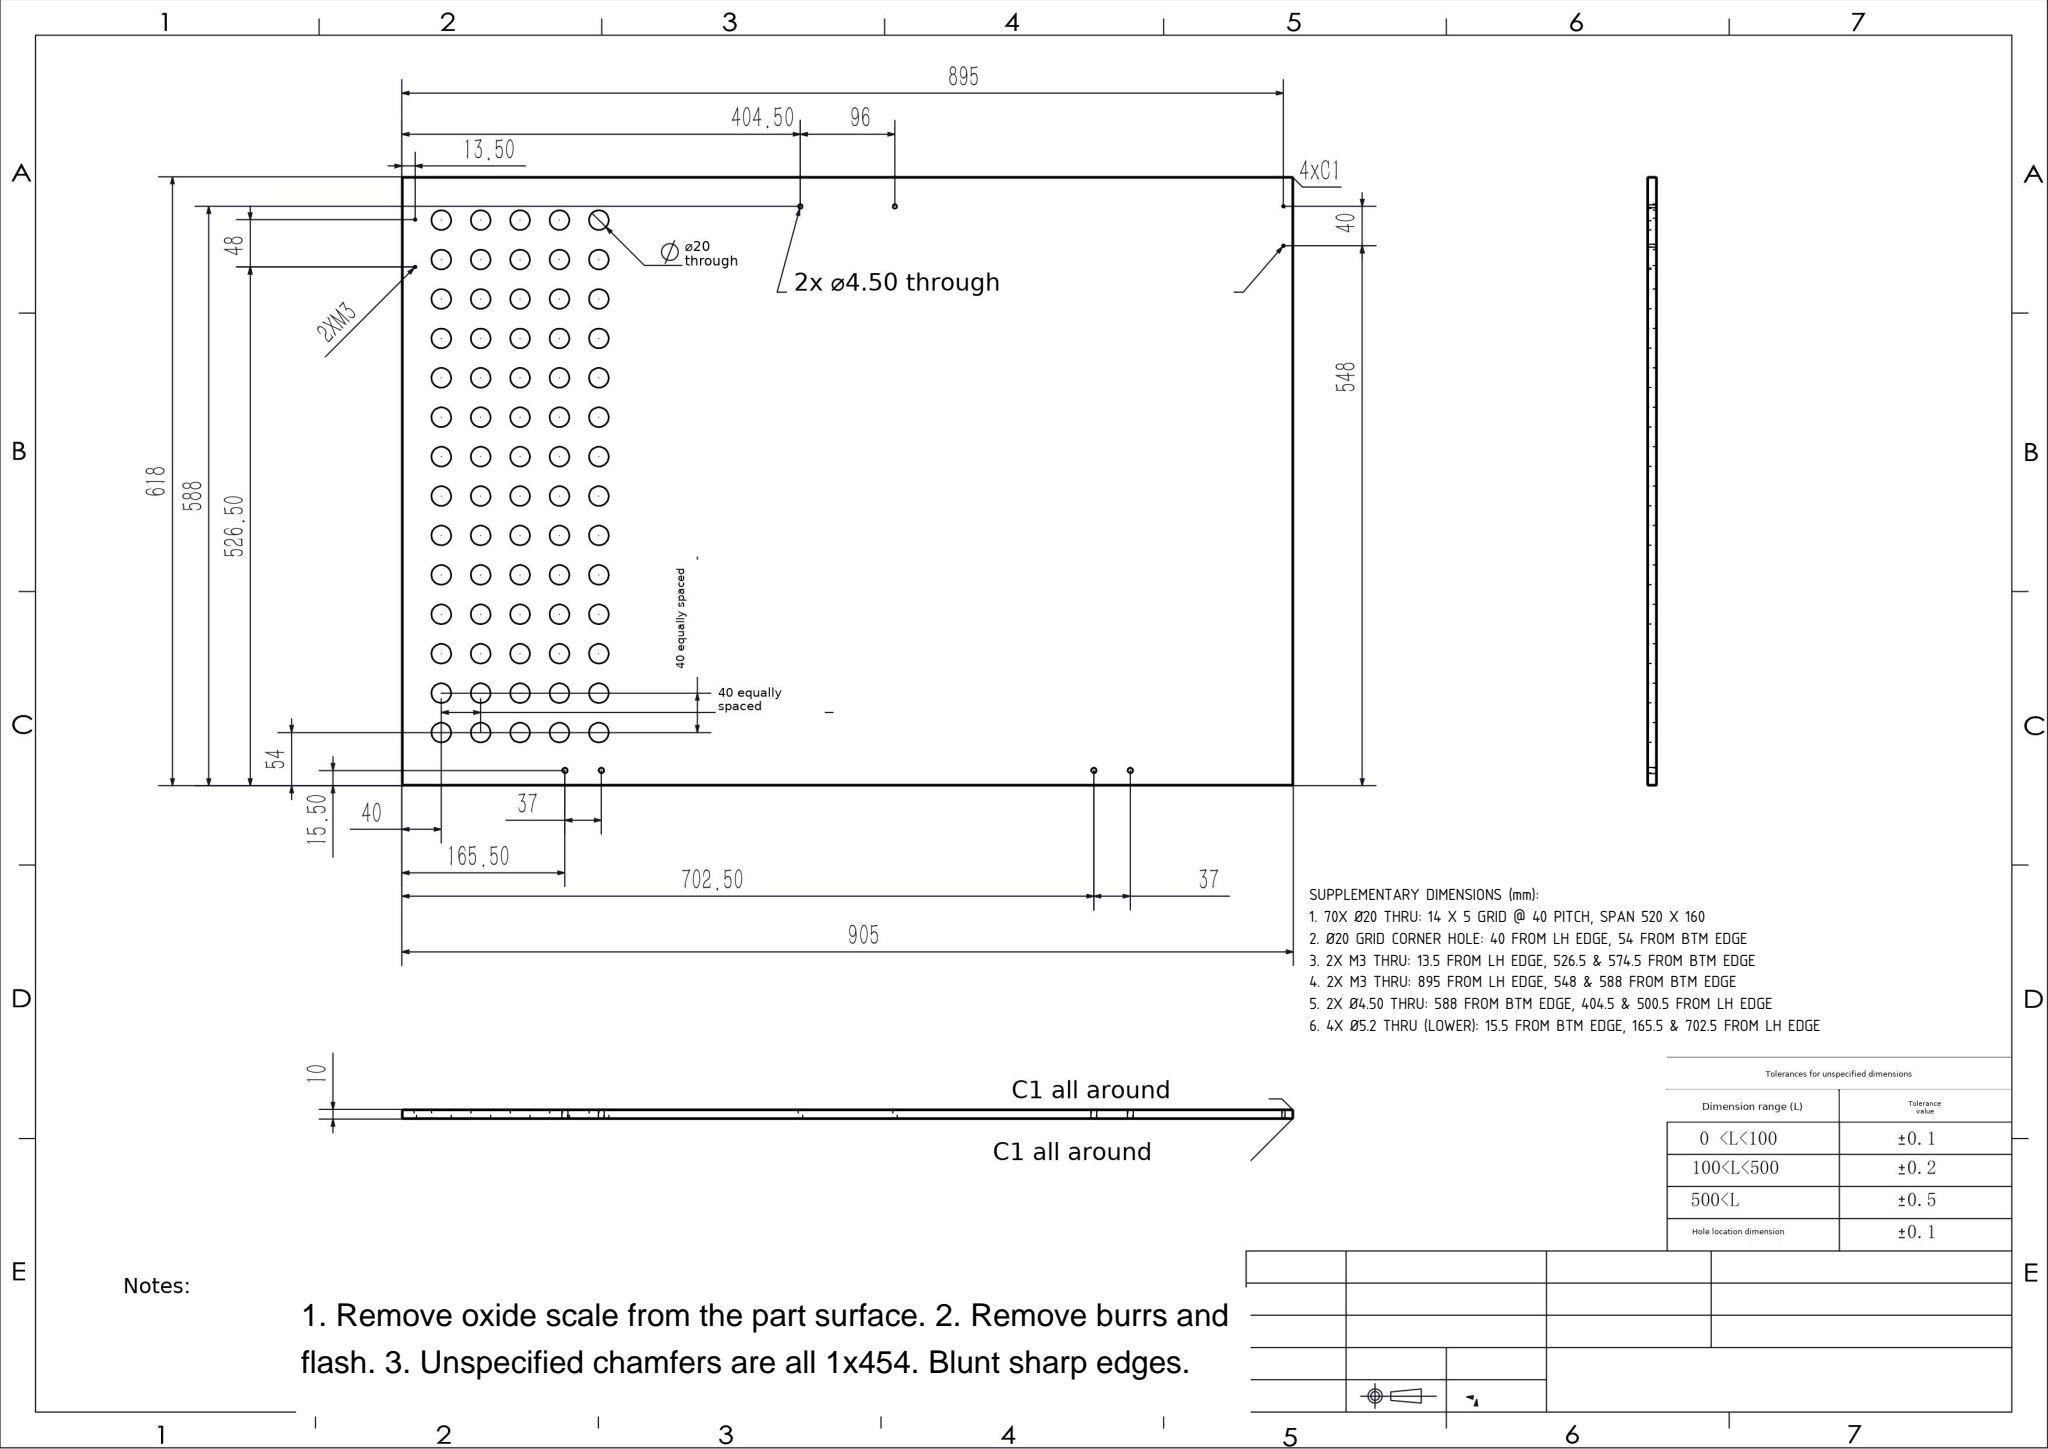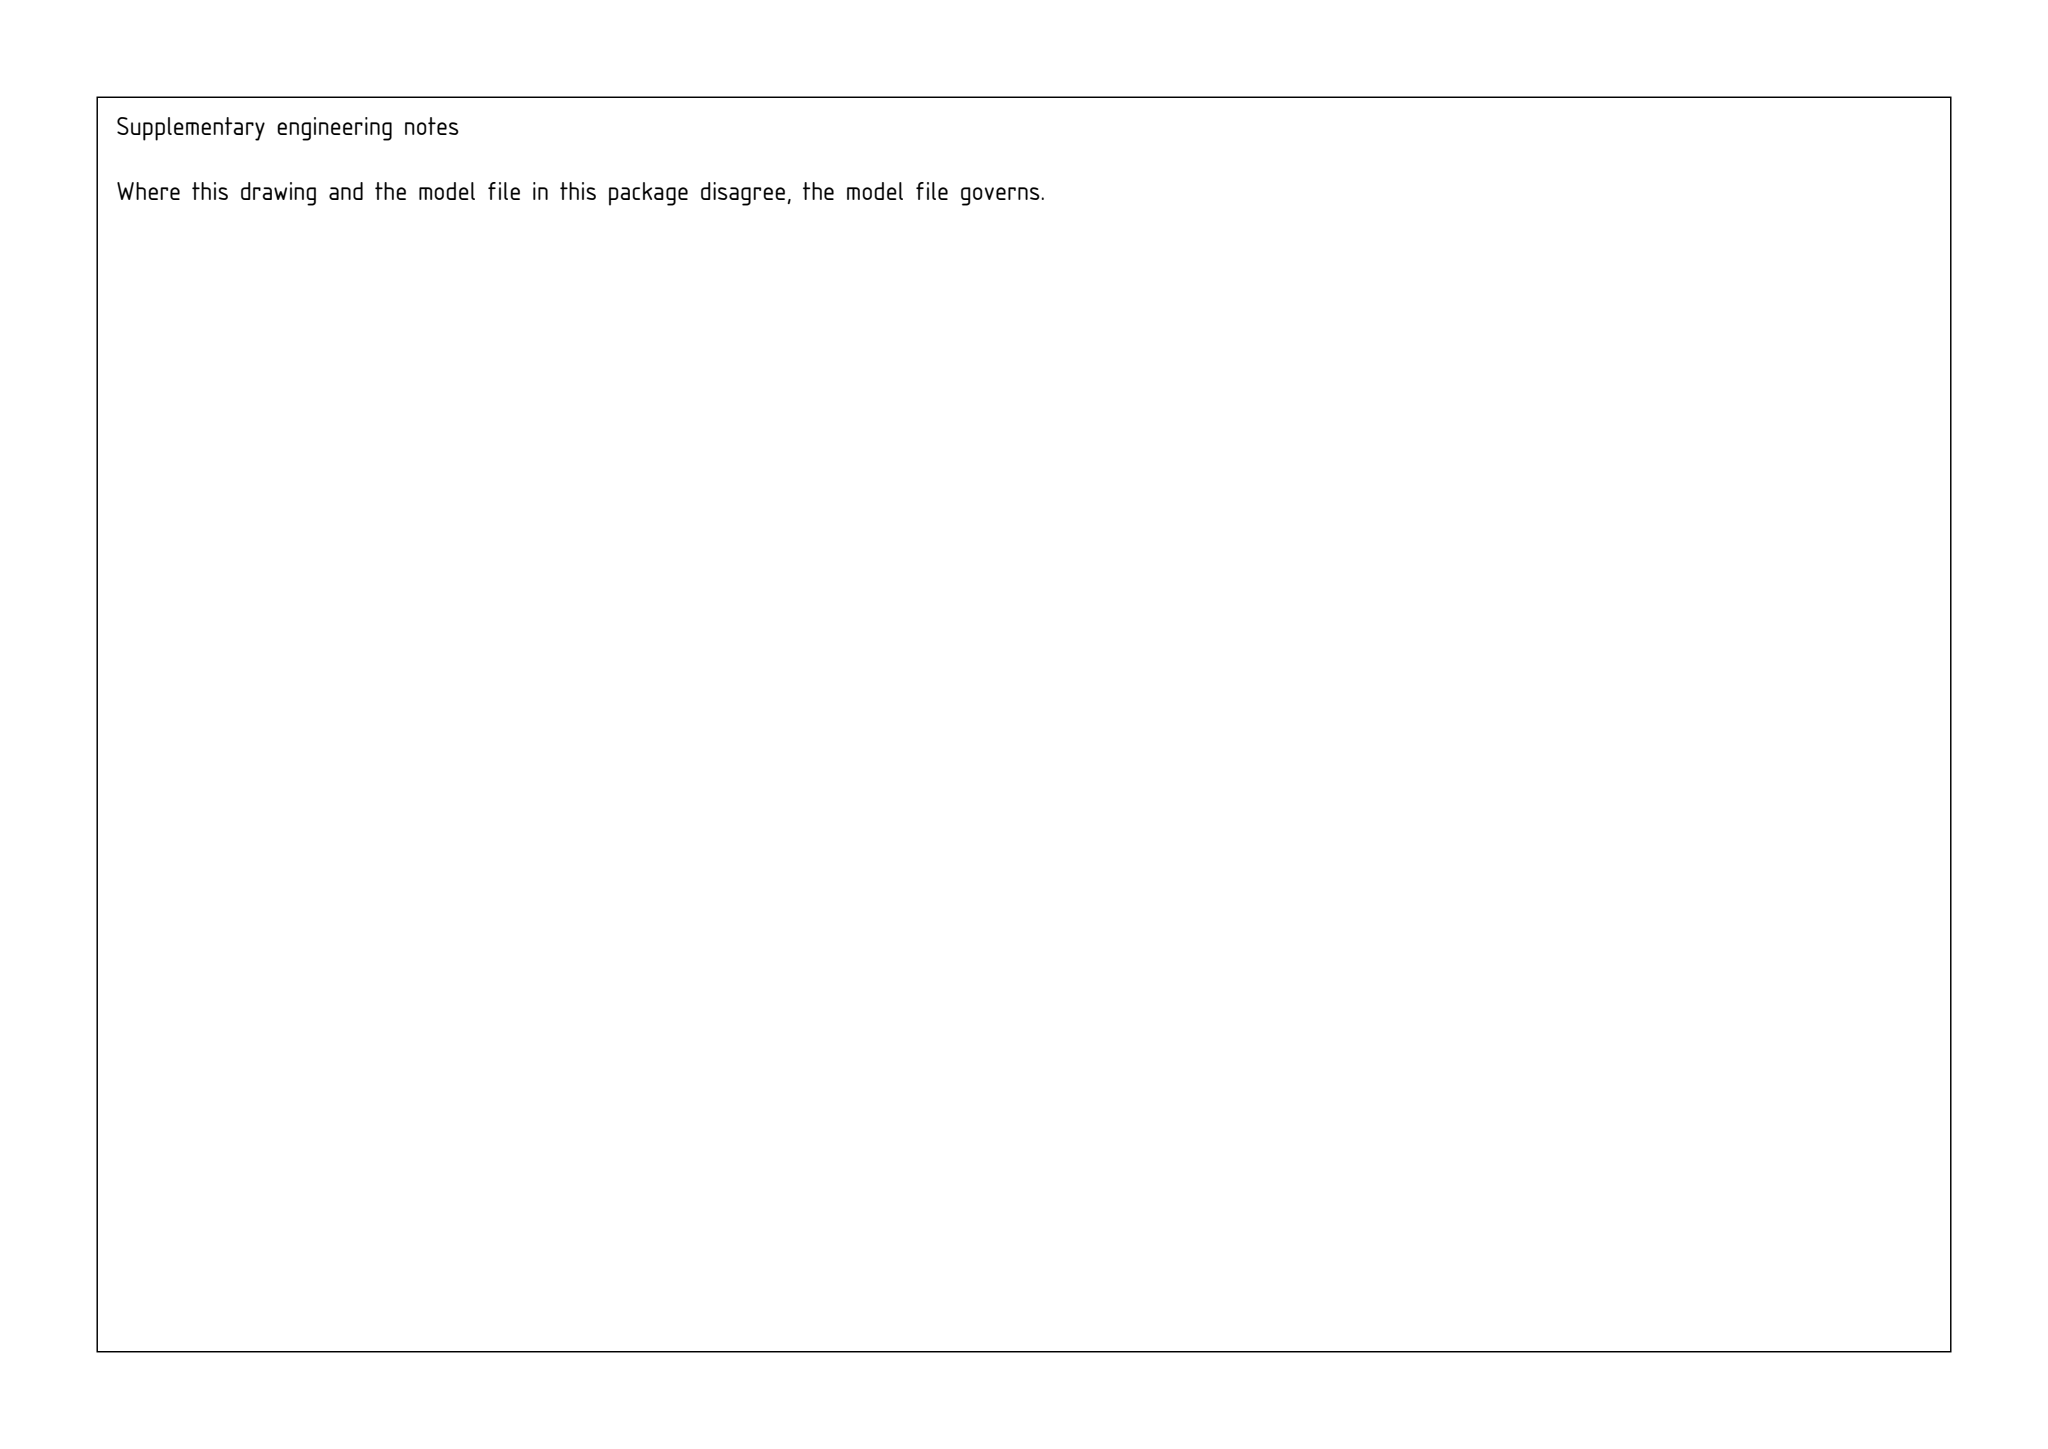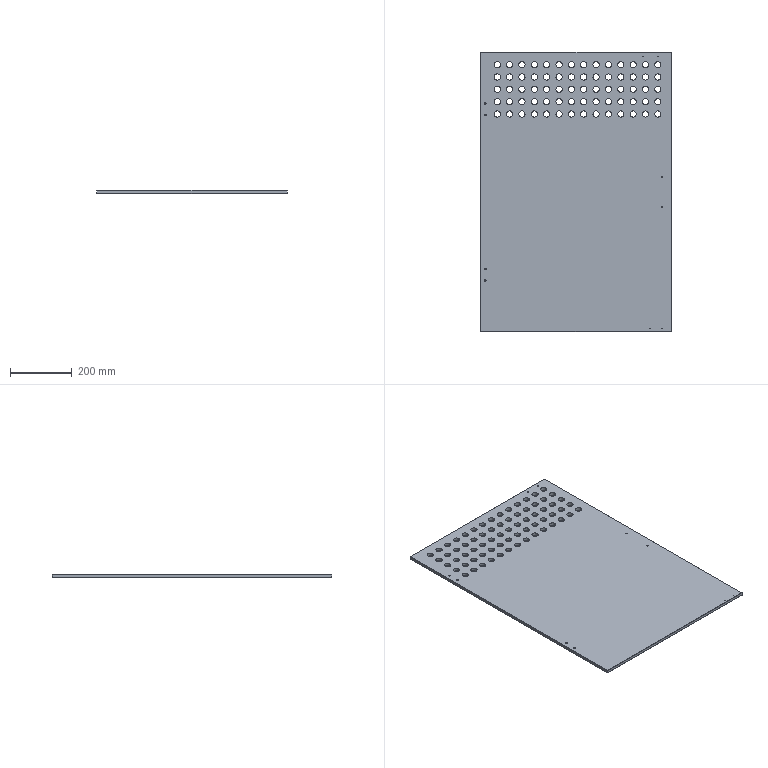Part | SolidWorks | mm | 1 solid | 186 faces | box 618 x 905 x 10 mm | volume 5368564 mm3 | cylinder 160 | plane 26 | commonest cylinder face diameters 20 x140 2.5 x8 5.2 x8 4.5 x4
build123d program:
from build123d import *

# Parameters (mm, degrees)
SKETCH1_W           = 618
SKETCH1_H           = 905
BOSS_EXTRUDE1_DEPTH = 5
CHAMFER1_SIZE       = 1
SKETCH2_R           = 2.6
CUT_EXTRUDE1_DEPTH  = 549.03
SKETCH3_R           = 2.25
CUT_EXTRUDE2_DEPTH  = 549.03
SKETCH4_R           = 1.25
CUT_EXTRUDE3_DEPTH  = 549.03
SKETCH6_R           = 10
CUT_EXTRUDE5_DEPTH  = 549.03
SKETCH7_R           = 1.25
CUT_EXTRUDE6_DEPTH  = 549.03


with BuildPart() as part:
    # Sketch1 → Boss-Extrude1 (new, symmetric)
    with BuildSketch(Plane.XY):
        Rectangle(SKETCH1_W, SKETCH1_H)
    extrude(amount=BOSS_EXTRUDE1_DEPTH, both=True)

    # Chamfer1
    chamfer1_edges = [part.edges().sort_by_distance(p)[0] for p in [
        (-309, 0, 5),
        (0, -452.5, 5),
        (309, 0, 5),
        (0, -452.5, -5),
        (-309, 0, -5),
        (0, 452.5, -5),
        (309, 0, -5),
        (0, 452.5, 5),
        (309, -452.5, 0),
        (-309, -452.5, 0),
        (-309, 452.5, 0),
        (309, 452.5, 0),
    ]]
    chamfer(chamfer1_edges, length=CHAMFER1_SIZE)

    # Sketch2 → Cut-Extrude1 (cut, through all)
    with BuildSketch(Plane.XY.offset(5)):
        with Locations((-293.5, 287)):
            Circle(SKETCH2_R)
        with Locations((-293.5, 250)):
            Circle(SKETCH2_R)
        with Locations(Location((-293.5, -250, 0), (0, 0, 180))):
            Circle(SKETCH2_R)
        with Locations(Location((-293.5, -287, 0), (0, 0, 180))):
            Circle(SKETCH2_R)
    extrude(amount=-CUT_EXTRUDE1_DEPTH, mode=Mode.SUBTRACT)

    # Sketch3 → Cut-Extrude2 (cut, through all)
    with BuildSketch(Plane.XY.offset(5)):
        with Locations((279, 48)):
            Circle(SKETCH3_R)
        with Locations((279, -48)):
            Circle(SKETCH3_R)
    extrude(amount=-CUT_EXTRUDE2_DEPTH, mode=Mode.SUBTRACT)

    # Sketch4 → Cut-Extrude3 (cut, through all)
    with BuildSketch(Plane.XY.offset(5)):
        with Locations((239, -442.5)):
            Circle(SKETCH4_R)
        with Locations((279, -442.5)):
            Circle(SKETCH4_R)
    extrude(amount=-CUT_EXTRUDE3_DEPTH, mode=Mode.SUBTRACT)

    # Sketch6 → Cut-Extrude5 (cut, through all)
    with BuildSketch(Plane(origin=(0, 0, -5), x_dir=(-1, 0, 0), z_dir=(0, 0, -1))):
        with Locations((-265, 412.5)):
            Circle(SKETCH6_R)
        with Locations((-225, 412.5)):
            Circle(SKETCH6_R)
        with Locations((-185, 412.5)):
            Circle(SKETCH6_R)
        with Locations((-145, 412.5)):
            Circle(SKETCH6_R)
        with Locations((-105, 412.5)):
            Circle(SKETCH6_R)
        with Locations((-65, 412.5)):
            Circle(SKETCH6_R)
        with Locations((-25, 412.5)):
            Circle(SKETCH6_R)
        with Locations((15, 412.5)):
            Circle(SKETCH6_R)
        with Locations((55, 412.5)):
            Circle(SKETCH6_R)
        with Locations((95, 412.5)):
            Circle(SKETCH6_R)
        with Locations((135, 412.5)):
            Circle(SKETCH6_R)
        with Locations((175, 412.5)):
            Circle(SKETCH6_R)
        with Locations((215, 412.5)):
            Circle(SKETCH6_R)
        with Locations((255, 412.5)):
            Circle(SKETCH6_R)
        with Locations((-225, 372.5)):
            Circle(SKETCH6_R)
        with Locations((-185, 372.5)):
            Circle(SKETCH6_R)
        with Locations((-145, 372.5)):
            Circle(SKETCH6_R)
        with Locations((-105, 372.5)):
            Circle(SKETCH6_R)
        with Locations((-65, 372.5)):
            Circle(SKETCH6_R)
        with Locations((-25, 372.5)):
            Circle(SKETCH6_R)
        with Locations((15, 372.5)):
            Circle(SKETCH6_R)
        with Locations((55, 372.5)):
            Circle(SKETCH6_R)
        with Locations((95, 372.5)):
            Circle(SKETCH6_R)
        with Locations((135, 372.5)):
            Circle(SKETCH6_R)
        with Locations((175, 372.5)):
            Circle(SKETCH6_R)
        with Locations((215, 372.5)):
            Circle(SKETCH6_R)
        with Locations((255, 372.5)):
            Circle(SKETCH6_R)
        with Locations((-225, 332.5)):
            Circle(SKETCH6_R)
        with Locations((-185, 332.5)):
            Circle(SKETCH6_R)
        with Locations((-145, 332.5)):
            Circle(SKETCH6_R)
        with Locations((-105, 332.5)):
            Circle(SKETCH6_R)
        with Locations((-65, 332.5)):
            Circle(SKETCH6_R)
        with Locations((-25, 332.5)):
            Circle(SKETCH6_R)
        with Locations((15, 332.5)):
            Circle(SKETCH6_R)
        with Locations((55, 332.5)):
            Circle(SKETCH6_R)
        with Locations((95, 332.5)):
            Circle(SKETCH6_R)
        with Locations((135, 332.5)):
            Circle(SKETCH6_R)
        with Locations((175, 332.5)):
            Circle(SKETCH6_R)
        with Locations((215, 332.5)):
            Circle(SKETCH6_R)
        with Locations((255, 332.5)):
            Circle(SKETCH6_R)
        with Locations((-225, 292.5)):
            Circle(SKETCH6_R)
        with Locations((-185, 292.5)):
            Circle(SKETCH6_R)
        with Locations((-145, 292.5)):
            Circle(SKETCH6_R)
        with Locations((-105, 292.5)):
            Circle(SKETCH6_R)
        with Locations((-65, 292.5)):
            Circle(SKETCH6_R)
        with Locations((-25, 292.5)):
            Circle(SKETCH6_R)
        with Locations((15, 292.5)):
            Circle(SKETCH6_R)
        with Locations((55, 292.5)):
            Circle(SKETCH6_R)
        with Locations((95, 292.5)):
            Circle(SKETCH6_R)
        with Locations((135, 292.5)):
            Circle(SKETCH6_R)
        with Locations((175, 292.5)):
            Circle(SKETCH6_R)
        with Locations((215, 292.5)):
            Circle(SKETCH6_R)
        with Locations((255, 292.5)):
            Circle(SKETCH6_R)
        with Locations((-225, 252.5)):
            Circle(SKETCH6_R)
        with Locations((-185, 252.5)):
            Circle(SKETCH6_R)
        with Locations((-145, 252.5)):
            Circle(SKETCH6_R)
        with Locations((-105, 252.5)):
            Circle(SKETCH6_R)
        with Locations((-65, 252.5)):
            Circle(SKETCH6_R)
        with Locations((-25, 252.5)):
            Circle(SKETCH6_R)
        with Locations((15, 252.5)):
            Circle(SKETCH6_R)
        with Locations((55, 252.5)):
            Circle(SKETCH6_R)
        with Locations((95, 252.5)):
            Circle(SKETCH6_R)
        with Locations((135, 252.5)):
            Circle(SKETCH6_R)
        with Locations((175, 252.5)):
            Circle(SKETCH6_R)
        with Locations((215, 252.5)):
            Circle(SKETCH6_R)
        with Locations((255, 252.5)):
            Circle(SKETCH6_R)
        with Locations((-265, 372.5)):
            Circle(SKETCH6_R)
        with Locations((-265, 332.5)):
            Circle(SKETCH6_R)
        with Locations((-265, 292.5)):
            Circle(SKETCH6_R)
        with Locations((-265, 252.5)):
            Circle(SKETCH6_R)
    extrude(amount=-CUT_EXTRUDE5_DEPTH, mode=Mode.SUBTRACT)

    # Sketch7 → Cut-Extrude6 (cut, through all)
    with BuildSketch(Plane.XY.offset(5)):
        with Locations((265.5, 439)):
            Circle(SKETCH7_R)
        with Locations((217.5, 439)):
            Circle(SKETCH7_R)
    extrude(amount=-CUT_EXTRUDE6_DEPTH, mode=Mode.SUBTRACT)


solid = part.part